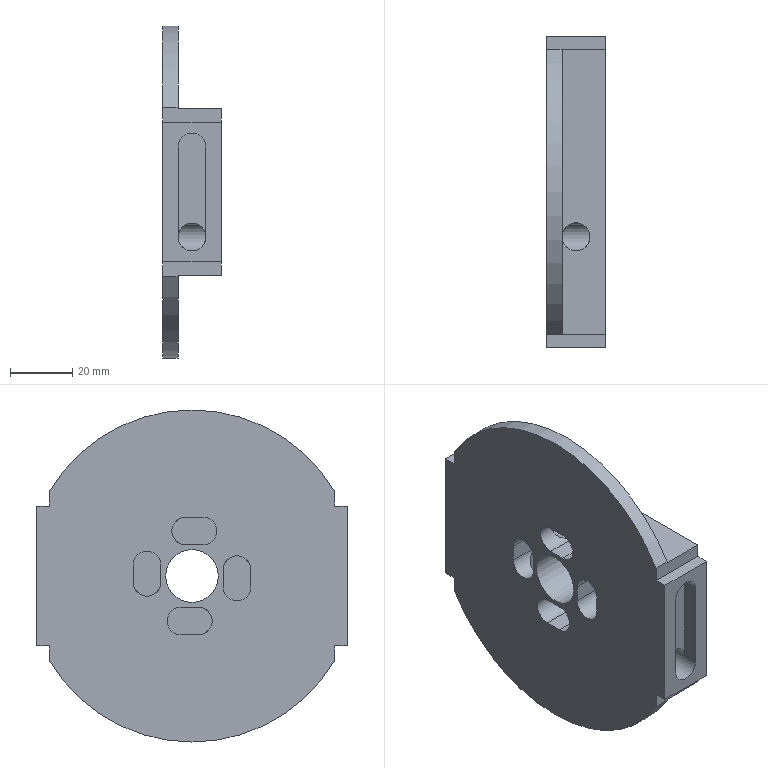Component | NX | INTERMEDIATE_FRAME | 1 solid | 59 faces | volume 97006 mm3 | plane 34 | cylinder 25 | commonest cylinder face diameters 9 x22 107 x2 17 x1